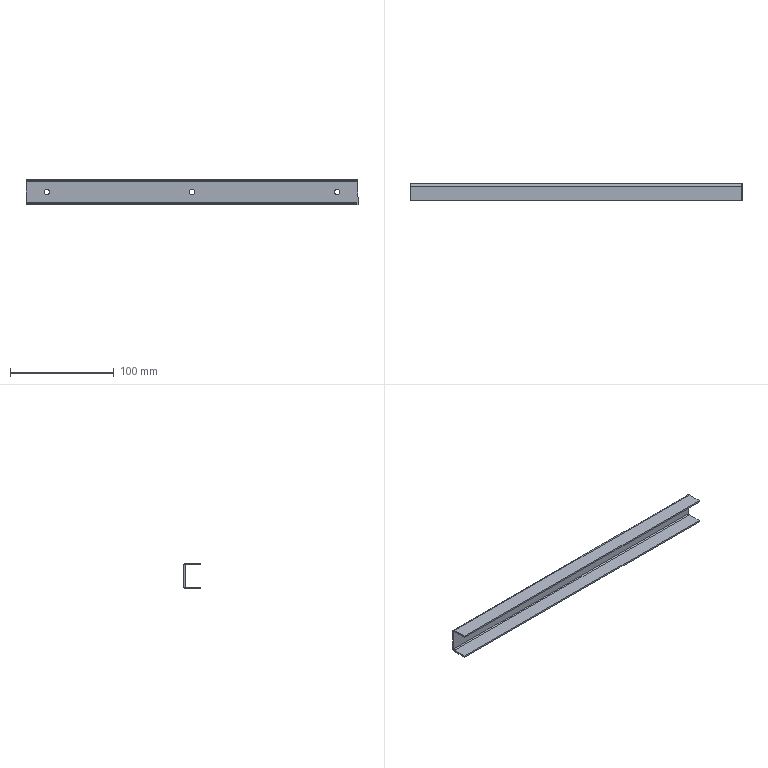Component | SolidWorks | GlassDoorAssembly-1_ShortBentPlate-5 | 1 solid | 28 faces | box 320 x 16 x 25 mm | volume 25103 mm3 | plane 18 | cylinder 10 | commonest cylinder face diameters 5.2 x6 5 x2 2 x2
STEP:
#1=CARTESIAN_POINT('',(-2.487,-19.472,-59.39));
#2=VERTEX_POINT('',#1);
#3=CARTESIAN_POINT('',(-2.283,-19.472,-59.39));
#4=VERTEX_POINT('',#3);
#5=CARTESIAN_POINT('',(-2.385,-19.472,-59.39));
#6=DIRECTION('',(0.,-1.,0.));
#7=DIRECTION('',(1.,0.,0.));
#8=AXIS2_PLACEMENT_3D('',#5,#6,#7);
#9=CIRCLE('',#8,0.1024);
#10=EDGE_CURVE('',#2,#4,#9,.T.);
#11=ORIENTED_EDGE('',*,*,#10,.T.);
#12=CARTESIAN_POINT('',(-2.283,-19.412,-59.39));
#13=VERTEX_POINT('',#12);
#14=CARTESIAN_POINT('',(-2.283,-19.491,-59.39));
#15=DIRECTION('',(-0.,1.,-0.));
#16=VECTOR('',#15,39.37);
#17=LINE('',#14,#16);
#18=EDGE_CURVE('',#4,#13,#17,.T.);
#19=ORIENTED_EDGE('',*,*,#18,.T.);
#20=CARTESIAN_POINT('',(-2.487,-19.412,-59.39));
#21=VERTEX_POINT('',#20);
#22=CARTESIAN_POINT('',(-2.385,-19.412,-59.39));
#23=DIRECTION('',(-0.,1.,-0.));
#24=DIRECTION('',(-1.,0.,0.));
#25=AXIS2_PLACEMENT_3D('',#22,#23,#24);
#26=CIRCLE('',#25,0.1024);
#27=EDGE_CURVE('',#13,#21,#26,.T.);
#28=ORIENTED_EDGE('',*,*,#27,.T.);
#29=CARTESIAN_POINT('',(-2.487,-19.491,-59.39));
#30=DIRECTION('',(-0.,1.,-0.));
#31=VECTOR('',#30,39.37);
#32=LINE('',#29,#31);
#33=EDGE_CURVE('',#2,#21,#32,.T.);
#34=ORIENTED_EDGE('',*,*,#33,.F.);
#35=EDGE_LOOP('',(#11,#19,#28,#34));
#36=FACE_OUTER_BOUND('',#35,.T.);
#37=CARTESIAN_POINT('',(-2.385,-19.491,-59.39));
#38=DIRECTION('',(-0.,1.,-0.));
#39=DIRECTION('',(-1.,0.,0.));
#40=AXIS2_PLACEMENT_3D('',#37,#38,#39);
#41=CYLINDRICAL_SURFACE('',#40,0.1024);
#42=ADVANCED_FACE('',(#36),#41,.F.);
#43=CARTESIAN_POINT('',(-13.511,-19.472,-59.39));
#44=VERTEX_POINT('',#43);
#45=CARTESIAN_POINT('',(-13.306,-19.472,-59.39));
#46=VERTEX_POINT('',#45);
#47=CARTESIAN_POINT('',(-13.409,-19.472,-59.39));
#48=DIRECTION('',(0.,-1.,0.));
#49=DIRECTION('',(1.,0.,0.));
#50=AXIS2_PLACEMENT_3D('',#47,#48,#49);
#51=CIRCLE('',#50,0.1024);
#52=EDGE_CURVE('',#44,#46,#51,.T.);
#53=ORIENTED_EDGE('',*,*,#52,.T.);
#54=CARTESIAN_POINT('',(-13.306,-19.412,-59.39));
#55=VERTEX_POINT('',#54);
#56=CARTESIAN_POINT('',(-13.306,-19.491,-59.39));
#57=DIRECTION('',(-0.,1.,-0.));
#58=VECTOR('',#57,39.37);
#59=LINE('',#56,#58);
#60=EDGE_CURVE('',#46,#55,#59,.T.);
#61=ORIENTED_EDGE('',*,*,#60,.T.);
#62=CARTESIAN_POINT('',(-13.511,-19.412,-59.39));
#63=VERTEX_POINT('',#62);
#64=CARTESIAN_POINT('',(-13.409,-19.412,-59.39));
#65=DIRECTION('',(-0.,1.,-0.));
#66=DIRECTION('',(-1.,0.,0.));
#67=AXIS2_PLACEMENT_3D('',#64,#65,#66);
#68=CIRCLE('',#67,0.1024);
#69=EDGE_CURVE('',#55,#63,#68,.T.);
#70=ORIENTED_EDGE('',*,*,#69,.T.);
#71=CARTESIAN_POINT('',(-13.511,-19.491,-59.39));
#72=DIRECTION('',(-0.,1.,-0.));
#73=VECTOR('',#72,39.37);
#74=LINE('',#71,#73);
#75=EDGE_CURVE('',#44,#63,#74,.T.);
#76=ORIENTED_EDGE('',*,*,#75,.F.);
#77=EDGE_LOOP('',(#53,#61,#70,#76));
#78=FACE_OUTER_BOUND('',#77,.T.);
#79=CARTESIAN_POINT('',(-13.409,-19.491,-59.39));
#80=DIRECTION('',(-0.,1.,-0.));
#81=DIRECTION('',(-1.,0.,0.));
#82=AXIS2_PLACEMENT_3D('',#79,#80,#81);
#83=CYLINDRICAL_SURFACE('',#82,0.1024);
#84=ADVANCED_FACE('',(#78),#83,.F.);
#85=CARTESIAN_POINT('',(-7.999,-19.472,-59.39));
#86=VERTEX_POINT('',#85);
#87=CARTESIAN_POINT('',(-7.794,-19.472,-59.39));
#88=VERTEX_POINT('',#87);
#89=CARTESIAN_POINT('',(-7.897,-19.472,-59.39));
#90=DIRECTION('',(0.,-1.,0.));
#91=DIRECTION('',(1.,0.,0.));
#92=AXIS2_PLACEMENT_3D('',#89,#90,#91);
#93=CIRCLE('',#92,0.1024);
#94=EDGE_CURVE('',#86,#88,#93,.T.);
#95=ORIENTED_EDGE('',*,*,#94,.T.);
#96=CARTESIAN_POINT('',(-7.794,-19.412,-59.39));
#97=VERTEX_POINT('',#96);
#98=CARTESIAN_POINT('',(-7.794,-19.491,-59.39));
#99=DIRECTION('',(-0.,1.,-0.));
#100=VECTOR('',#99,39.37);
#101=LINE('',#98,#100);
#102=EDGE_CURVE('',#88,#97,#101,.T.);
#103=ORIENTED_EDGE('',*,*,#102,.T.);
#104=CARTESIAN_POINT('',(-7.999,-19.412,-59.39));
#105=VERTEX_POINT('',#104);
#106=CARTESIAN_POINT('',(-7.897,-19.412,-59.39));
#107=DIRECTION('',(-0.,1.,-0.));
#108=DIRECTION('',(-1.,0.,0.));
#109=AXIS2_PLACEMENT_3D('',#106,#107,#108);
#110=CIRCLE('',#109,0.1024);
#111=EDGE_CURVE('',#97,#105,#110,.T.);
#112=ORIENTED_EDGE('',*,*,#111,.T.);
#113=CARTESIAN_POINT('',(-7.999,-19.491,-59.39));
#114=DIRECTION('',(-0.,1.,-0.));
#115=VECTOR('',#114,39.37);
#116=LINE('',#113,#115);
#117=EDGE_CURVE('',#86,#105,#116,.T.);
#118=ORIENTED_EDGE('',*,*,#117,.F.);
#119=EDGE_LOOP('',(#95,#103,#112,#118));
#120=FACE_OUTER_BOUND('',#119,.T.);
#121=CARTESIAN_POINT('',(-7.897,-19.491,-59.39));
#122=DIRECTION('',(-0.,1.,-0.));
#123=DIRECTION('',(-1.,0.,0.));
#124=AXIS2_PLACEMENT_3D('',#121,#122,#123);
#125=CYLINDRICAL_SURFACE('',#124,0.1024);
#126=ADVANCED_FACE('',(#120),#125,.F.);
#127=CARTESIAN_POINT('',(-2.385,-19.412,-59.39));
#128=DIRECTION('',(-0.,1.,-0.));
#129=DIRECTION('',(-1.,0.,0.));
#130=AXIS2_PLACEMENT_3D('',#127,#128,#129);
#131=CIRCLE('',#130,0.1024);
#132=EDGE_CURVE('',#21,#13,#131,.T.);
#133=ORIENTED_EDGE('',*,*,#132,.F.);
#134=ORIENTED_EDGE('',*,*,#27,.F.);
#135=EDGE_LOOP('',(#133,#134));
#136=FACE_BOUND('',#135,.T.);
#137=CARTESIAN_POINT('',(-13.409,-19.412,-59.39));
#138=DIRECTION('',(-0.,1.,-0.));
#139=DIRECTION('',(-1.,0.,0.));
#140=AXIS2_PLACEMENT_3D('',#137,#138,#139);
#141=CIRCLE('',#140,0.1024);
#142=EDGE_CURVE('',#63,#55,#141,.T.);
#143=ORIENTED_EDGE('',*,*,#142,.F.);
#144=ORIENTED_EDGE('',*,*,#69,.F.);
#145=EDGE_LOOP('',(#143,#144));
#146=FACE_BOUND('',#145,.T.);
#147=CARTESIAN_POINT('',(-7.897,-19.412,-59.39));
#148=DIRECTION('',(-0.,1.,-0.));
#149=DIRECTION('',(-1.,0.,0.));
#150=AXIS2_PLACEMENT_3D('',#147,#148,#149);
#151=CIRCLE('',#150,0.1024);
#152=EDGE_CURVE('',#105,#97,#151,.T.);
#153=ORIENTED_EDGE('',*,*,#152,.F.);
#154=ORIENTED_EDGE('',*,*,#111,.F.);
#155=EDGE_LOOP('',(#153,#154));
#156=FACE_BOUND('',#155,.T.);
#157=CARTESIAN_POINT('',(-14.196,-19.412,-58.996));
#158=VERTEX_POINT('',#157);
#159=CARTESIAN_POINT('',(-1.598,-19.412,-58.996));
#160=VERTEX_POINT('',#159);
#161=CARTESIAN_POINT('',(-14.196,-19.412,-58.996));
#162=DIRECTION('',(1.,0.,0.));
#163=VECTOR('',#162,39.37);
#164=LINE('',#161,#163);
#165=EDGE_CURVE('',#158,#160,#164,.T.);
#166=ORIENTED_EDGE('',*,*,#165,.T.);
#167=CARTESIAN_POINT('',(-1.598,-19.412,-59.783));
#168=VERTEX_POINT('',#167);
#169=CARTESIAN_POINT('',(-1.598,-19.412,-58.898));
#170=DIRECTION('',(-0.,0.,1.));
#171=VECTOR('',#170,39.37);
#172=LINE('',#169,#171);
#173=EDGE_CURVE('',#168,#160,#172,.T.);
#174=ORIENTED_EDGE('',*,*,#173,.F.);
#175=CARTESIAN_POINT('',(-14.196,-19.412,-59.783));
#176=VERTEX_POINT('',#175);
#177=CARTESIAN_POINT('',(-1.598,-19.412,-59.783));
#178=DIRECTION('',(-1.,-0.,-0.));
#179=VECTOR('',#178,39.37);
#180=LINE('',#177,#179);
#181=EDGE_CURVE('',#168,#176,#180,.T.);
#182=ORIENTED_EDGE('',*,*,#181,.T.);
#183=CARTESIAN_POINT('',(-14.196,-19.412,-58.898));
#184=DIRECTION('',(0.,-0.,-1.));
#185=VECTOR('',#184,39.37);
#186=LINE('',#183,#185);
#187=EDGE_CURVE('',#158,#176,#186,.T.);
#188=ORIENTED_EDGE('',*,*,#187,.F.);
#189=EDGE_LOOP('',(#166,#174,#182,#188));
#190=FACE_OUTER_BOUND('',#189,.T.);
#191=CARTESIAN_POINT('',(-1.598,-19.412,-59.882));
#192=DIRECTION('',(0.,-1.,0.));
#193=DIRECTION('',(1.,0.,0.));
#194=AXIS2_PLACEMENT_3D('',#191,#192,#193);
#195=PLANE('',#194);
#196=ADVANCED_FACE('',(#136,#146,#156,#190),#195,.F.);
#197=ORIENTED_EDGE('',*,*,#10,.F.);
#198=CARTESIAN_POINT('',(-2.385,-19.472,-59.39));
#199=DIRECTION('',(0.,-1.,0.));
#200=DIRECTION('',(1.,0.,0.));
#201=AXIS2_PLACEMENT_3D('',#198,#199,#200);
#202=CIRCLE('',#201,0.1024);
#203=EDGE_CURVE('',#4,#2,#202,.T.);
#204=ORIENTED_EDGE('',*,*,#203,.F.);
#205=EDGE_LOOP('',(#197,#204));
#206=FACE_BOUND('',#205,.T.);
#207=ORIENTED_EDGE('',*,*,#52,.F.);
#208=CARTESIAN_POINT('',(-13.409,-19.472,-59.39));
#209=DIRECTION('',(0.,-1.,0.));
#210=DIRECTION('',(1.,0.,0.));
#211=AXIS2_PLACEMENT_3D('',#208,#209,#210);
#212=CIRCLE('',#211,0.1024);
#213=EDGE_CURVE('',#46,#44,#212,.T.);
#214=ORIENTED_EDGE('',*,*,#213,.F.);
#215=EDGE_LOOP('',(#207,#214));
#216=FACE_BOUND('',#215,.T.);
#217=ORIENTED_EDGE('',*,*,#94,.F.);
#218=CARTESIAN_POINT('',(-7.897,-19.472,-59.39));
#219=DIRECTION('',(0.,-1.,0.));
#220=DIRECTION('',(1.,0.,0.));
#221=AXIS2_PLACEMENT_3D('',#218,#219,#220);
#222=CIRCLE('',#221,0.1024);
#223=EDGE_CURVE('',#88,#86,#222,.T.);
#224=ORIENTED_EDGE('',*,*,#223,.F.);
#225=EDGE_LOOP('',(#217,#224));
#226=FACE_BOUND('',#225,.T.);
#227=CARTESIAN_POINT('',(-1.598,-19.472,-59.783));
#228=VERTEX_POINT('',#227);
#229=CARTESIAN_POINT('',(-1.598,-19.472,-58.996));
#230=VERTEX_POINT('',#229);
#231=CARTESIAN_POINT('',(-1.598,-19.472,-58.898));
#232=DIRECTION('',(-0.,0.,1.));
#233=VECTOR('',#232,39.37);
#234=LINE('',#231,#233);
#235=EDGE_CURVE('',#228,#230,#234,.T.);
#236=ORIENTED_EDGE('',*,*,#235,.T.);
#237=CARTESIAN_POINT('',(-14.196,-19.472,-58.996));
#238=VERTEX_POINT('',#237);
#239=CARTESIAN_POINT('',(-14.196,-19.472,-58.996));
#240=DIRECTION('',(1.,0.,0.));
#241=VECTOR('',#240,39.37);
#242=LINE('',#239,#241);
#243=EDGE_CURVE('',#238,#230,#242,.T.);
#244=ORIENTED_EDGE('',*,*,#243,.F.);
#245=CARTESIAN_POINT('',(-14.196,-19.472,-59.783));
#246=VERTEX_POINT('',#245);
#247=CARTESIAN_POINT('',(-14.196,-19.472,-58.898));
#248=DIRECTION('',(0.,-0.,-1.));
#249=VECTOR('',#248,39.37);
#250=LINE('',#247,#249);
#251=EDGE_CURVE('',#238,#246,#250,.T.);
#252=ORIENTED_EDGE('',*,*,#251,.T.);
#253=CARTESIAN_POINT('',(-1.598,-19.472,-59.783));
#254=DIRECTION('',(-1.,-0.,-0.));
#255=VECTOR('',#254,39.37);
#256=LINE('',#253,#255);
#257=EDGE_CURVE('',#228,#246,#256,.T.);
#258=ORIENTED_EDGE('',*,*,#257,.F.);
#259=EDGE_LOOP('',(#236,#244,#252,#258));
#260=FACE_OUTER_BOUND('',#259,.T.);
#261=CARTESIAN_POINT('',(-1.598,-19.472,-59.882));
#262=DIRECTION('',(0.,-1.,0.));
#263=DIRECTION('',(1.,0.,0.));
#264=AXIS2_PLACEMENT_3D('',#261,#262,#263);
#265=PLANE('',#264);
#266=ADVANCED_FACE('',(#206,#216,#226,#260),#265,.T.);
#267=ORIENTED_EDGE('',*,*,#251,.F.);
#268=CARTESIAN_POINT('',(-14.196,-19.472,-58.996));
#269=DIRECTION('',(-0.,1.,-0.));
#270=VECTOR('',#269,39.37);
#271=LINE('',#268,#270);
#272=EDGE_CURVE('',#238,#158,#271,.T.);
#273=ORIENTED_EDGE('',*,*,#272,.T.);
#274=ORIENTED_EDGE('',*,*,#187,.T.);
#275=CARTESIAN_POINT('',(-14.196,-19.472,-59.783));
#276=DIRECTION('',(-0.,1.,-0.));
#277=VECTOR('',#276,39.37);
#278=LINE('',#275,#277);
#279=EDGE_CURVE('',#246,#176,#278,.T.);
#280=ORIENTED_EDGE('',*,*,#279,.F.);
#281=EDGE_LOOP('',(#267,#273,#274,#280));
#282=FACE_OUTER_BOUND('',#281,.T.);
#283=CARTESIAN_POINT('',(-14.196,-19.412,-58.898));
#284=DIRECTION('',(-1.,-0.,-0.));
#285=DIRECTION('',(0.,-1.,0.));
#286=AXIS2_PLACEMENT_3D('',#283,#284,#285);
#287=PLANE('',#286);
#288=ADVANCED_FACE('',(#282),#287,.T.);
#289=CARTESIAN_POINT('',(-1.598,-19.472,-58.996));
#290=DIRECTION('',(-0.,1.,-0.));
#291=VECTOR('',#290,39.37);
#292=LINE('',#289,#291);
#293=EDGE_CURVE('',#230,#160,#292,.T.);
#294=ORIENTED_EDGE('',*,*,#293,.F.);
#295=ORIENTED_EDGE('',*,*,#235,.F.);
#296=CARTESIAN_POINT('',(-1.598,-19.472,-59.783));
#297=DIRECTION('',(-0.,1.,-0.));
#298=VECTOR('',#297,39.37);
#299=LINE('',#296,#298);
#300=EDGE_CURVE('',#228,#168,#299,.T.);
#301=ORIENTED_EDGE('',*,*,#300,.T.);
#302=ORIENTED_EDGE('',*,*,#173,.T.);
#303=EDGE_LOOP('',(#294,#295,#301,#302));
#304=FACE_OUTER_BOUND('',#303,.T.);
#305=CARTESIAN_POINT('',(-1.598,-19.412,-58.898));
#306=DIRECTION('',(1.,0.,0.));
#307=DIRECTION('',(-0.,1.,-0.));
#308=AXIS2_PLACEMENT_3D('',#305,#306,#307);
#309=PLANE('',#308);
#310=ADVANCED_FACE('',(#304),#309,.T.);
#311=CARTESIAN_POINT('',(-14.196,-19.511,-59.823));
#312=VERTEX_POINT('',#311);
#313=CARTESIAN_POINT('',(-14.196,-19.511,-59.882));
#314=VERTEX_POINT('',#313);
#315=CARTESIAN_POINT('',(-14.196,-19.511,-59.882));
#316=DIRECTION('',(0.,0.,-1.));
#317=VECTOR('',#316,39.37);
#318=LINE('',#315,#317);
#319=EDGE_CURVE('',#312,#314,#318,.T.);
#320=ORIENTED_EDGE('',*,*,#319,.F.);
#321=CARTESIAN_POINT('',(-14.196,-19.511,-59.783));
#322=DIRECTION('',(-1.,-0.,-0.));
#323=DIRECTION('',(0.,1.,0.));
#324=AXIS2_PLACEMENT_3D('',#321,#322,#323);
#325=CIRCLE('',#324,0.03937);
#326=EDGE_CURVE('',#246,#312,#325,.T.);
#327=ORIENTED_EDGE('',*,*,#326,.F.);
#328=ORIENTED_EDGE('',*,*,#279,.T.);
#329=CARTESIAN_POINT('',(-14.196,-19.511,-59.783));
#330=DIRECTION('',(-1.,-0.,-0.));
#331=DIRECTION('',(0.,1.,0.));
#332=AXIS2_PLACEMENT_3D('',#329,#330,#331);
#333=CIRCLE('',#332,0.09843);
#334=EDGE_CURVE('',#176,#314,#333,.T.);
#335=ORIENTED_EDGE('',*,*,#334,.T.);
#336=EDGE_LOOP('',(#320,#327,#328,#335));
#337=FACE_OUTER_BOUND('',#336,.T.);
#338=CARTESIAN_POINT('',(-14.196,-19.511,-59.783));
#339=DIRECTION('',(-1.,-0.,-0.));
#340=DIRECTION('',(0.,-1.,0.));
#341=AXIS2_PLACEMENT_3D('',#338,#339,#340);
#342=PLANE('',#341);
#343=ADVANCED_FACE('',(#337),#342,.T.);
#344=CARTESIAN_POINT('',(-1.598,-19.511,-59.823));
#345=VERTEX_POINT('',#344);
#346=CARTESIAN_POINT('',(-1.598,-19.511,-59.783));
#347=DIRECTION('',(1.,0.,0.));
#348=DIRECTION('',(0.,1.,0.));
#349=AXIS2_PLACEMENT_3D('',#346,#347,#348);
#350=CIRCLE('',#349,0.03937);
#351=EDGE_CURVE('',#345,#228,#350,.T.);
#352=ORIENTED_EDGE('',*,*,#351,.F.);
#353=CARTESIAN_POINT('',(-1.598,-19.511,-59.882));
#354=VERTEX_POINT('',#353);
#355=CARTESIAN_POINT('',(-1.598,-19.511,-59.823));
#356=DIRECTION('',(0.,0.,-1.));
#357=VECTOR('',#356,39.37);
#358=LINE('',#355,#357);
#359=EDGE_CURVE('',#345,#354,#358,.T.);
#360=ORIENTED_EDGE('',*,*,#359,.T.);
#361=CARTESIAN_POINT('',(-1.598,-19.511,-59.783));
#362=DIRECTION('',(1.,0.,0.));
#363=DIRECTION('',(0.,1.,0.));
#364=AXIS2_PLACEMENT_3D('',#361,#362,#363);
#365=CIRCLE('',#364,0.09843);
#366=EDGE_CURVE('',#354,#168,#365,.T.);
#367=ORIENTED_EDGE('',*,*,#366,.T.);
#368=ORIENTED_EDGE('',*,*,#300,.F.);
#369=EDGE_LOOP('',(#352,#360,#367,#368));
#370=FACE_OUTER_BOUND('',#369,.T.);
#371=CARTESIAN_POINT('',(-1.598,-19.511,-59.783));
#372=DIRECTION('',(-1.,-0.,-0.));
#373=DIRECTION('',(0.,-1.,0.));
#374=AXIS2_PLACEMENT_3D('',#371,#372,#373);
#375=PLANE('',#374);
#376=ADVANCED_FACE('',(#370),#375,.F.);
#377=ORIENTED_EDGE('',*,*,#181,.F.);
#378=ORIENTED_EDGE('',*,*,#366,.F.);
#379=CARTESIAN_POINT('',(-14.196,-19.511,-59.882));
#380=DIRECTION('',(-1.,-0.,-0.));
#381=VECTOR('',#380,39.37);
#382=LINE('',#379,#381);
#383=EDGE_CURVE('',#354,#314,#382,.T.);
#384=ORIENTED_EDGE('',*,*,#383,.T.);
#385=ORIENTED_EDGE('',*,*,#334,.F.);
#386=EDGE_LOOP('',(#377,#378,#384,#385));
#387=FACE_OUTER_BOUND('',#386,.T.);
#388=CARTESIAN_POINT('',(-1.598,-19.511,-59.783));
#389=DIRECTION('',(1.,0.,0.));
#390=DIRECTION('',(0.,0.,-1.));
#391=AXIS2_PLACEMENT_3D('',#388,#389,#390);
#392=CYLINDRICAL_SURFACE('',#391,0.09843);
#393=ADVANCED_FACE('',(#387),#392,.T.);
#394=ORIENTED_EDGE('',*,*,#257,.T.);
#395=ORIENTED_EDGE('',*,*,#326,.T.);
#396=CARTESIAN_POINT('',(-14.196,-19.511,-59.823));
#397=DIRECTION('',(1.,0.,0.));
#398=VECTOR('',#397,39.37);
#399=LINE('',#396,#398);
#400=EDGE_CURVE('',#312,#345,#399,.T.);
#401=ORIENTED_EDGE('',*,*,#400,.T.);
#402=ORIENTED_EDGE('',*,*,#351,.T.);
#403=EDGE_LOOP('',(#394,#395,#401,#402));
#404=FACE_OUTER_BOUND('',#403,.T.);
#405=CARTESIAN_POINT('',(-1.598,-19.511,-59.783));
#406=DIRECTION('',(1.,0.,0.));
#407=DIRECTION('',(0.,0.,-1.));
#408=AXIS2_PLACEMENT_3D('',#405,#406,#407);
#409=CYLINDRICAL_SURFACE('',#408,0.03937);
#410=ADVANCED_FACE('',(#404),#409,.F.);
#411=ORIENTED_EDGE('',*,*,#319,.T.);
#412=CARTESIAN_POINT('',(-14.196,-20.042,-59.882));
#413=VERTEX_POINT('',#412);
#414=CARTESIAN_POINT('',(-14.196,-20.042,-59.882));
#415=DIRECTION('',(-0.,1.,0.));
#416=VECTOR('',#415,39.37);
#417=LINE('',#414,#416);
#418=EDGE_CURVE('',#413,#314,#417,.T.);
#419=ORIENTED_EDGE('',*,*,#418,.F.);
#420=CARTESIAN_POINT('',(-14.196,-20.042,-59.823));
#421=VERTEX_POINT('',#420);
#422=CARTESIAN_POINT('',(-14.196,-20.042,-59.882));
#423=DIRECTION('',(-0.,-0.,1.));
#424=VECTOR('',#423,39.37);
#425=LINE('',#422,#424);
#426=EDGE_CURVE('',#413,#421,#425,.T.);
#427=ORIENTED_EDGE('',*,*,#426,.T.);
#428=CARTESIAN_POINT('',(-14.196,-19.472,-59.823));
#429=DIRECTION('',(-0.,1.,0.));
#430=VECTOR('',#429,39.37);
#431=LINE('',#428,#430);
#432=EDGE_CURVE('',#421,#312,#431,.T.);
#433=ORIENTED_EDGE('',*,*,#432,.T.);
#434=EDGE_LOOP('',(#411,#419,#427,#433));
#435=FACE_OUTER_BOUND('',#434,.T.);
#436=CARTESIAN_POINT('',(-14.196,-19.472,-59.882));
#437=DIRECTION('',(1.,0.,0.));
#438=DIRECTION('',(-0.,1.,-0.));
#439=AXIS2_PLACEMENT_3D('',#436,#437,#438);
#440=PLANE('',#439);
#441=ADVANCED_FACE('',(#435),#440,.F.);
#442=ORIENTED_EDGE('',*,*,#359,.F.);
#443=CARTESIAN_POINT('',(-1.598,-20.042,-59.823));
#444=VERTEX_POINT('',#443);
#445=CARTESIAN_POINT('',(-1.598,-20.042,-59.823));
#446=DIRECTION('',(0.,-1.,-0.));
#447=VECTOR('',#446,39.37);
#448=LINE('',#445,#447);
#449=EDGE_CURVE('',#345,#444,#448,.T.);
#450=ORIENTED_EDGE('',*,*,#449,.T.);
#451=CARTESIAN_POINT('',(-1.598,-20.042,-59.882));
#452=VERTEX_POINT('',#451);
#453=CARTESIAN_POINT('',(-1.598,-20.042,-59.882));
#454=DIRECTION('',(-0.,-0.,1.));
#455=VECTOR('',#454,39.37);
#456=LINE('',#453,#455);
#457=EDGE_CURVE('',#452,#444,#456,.T.);
#458=ORIENTED_EDGE('',*,*,#457,.F.);
#459=CARTESIAN_POINT('',(-1.598,-20.042,-59.882));
#460=DIRECTION('',(0.,-1.,-0.));
#461=VECTOR('',#460,39.37);
#462=LINE('',#459,#461);
#463=EDGE_CURVE('',#354,#452,#462,.T.);
#464=ORIENTED_EDGE('',*,*,#463,.F.);
#465=EDGE_LOOP('',(#442,#450,#458,#464));
#466=FACE_OUTER_BOUND('',#465,.T.);
#467=CARTESIAN_POINT('',(-1.598,-20.042,-59.882));
#468=DIRECTION('',(-1.,-0.,-0.));
#469=DIRECTION('',(0.,-1.,0.));
#470=AXIS2_PLACEMENT_3D('',#467,#468,#469);
#471=PLANE('',#470);
#472=ADVANCED_FACE('',(#466),#471,.F.);
#473=ORIENTED_EDGE('',*,*,#383,.F.);
#474=ORIENTED_EDGE('',*,*,#463,.T.);
#475=CARTESIAN_POINT('',(-14.196,-20.042,-59.882));
#476=DIRECTION('',(-1.,-0.,-0.));
#477=VECTOR('',#476,39.37);
#478=LINE('',#475,#477);
#479=EDGE_CURVE('',#452,#413,#478,.T.);
#480=ORIENTED_EDGE('',*,*,#479,.T.);
#481=ORIENTED_EDGE('',*,*,#418,.T.);
#482=EDGE_LOOP('',(#473,#474,#480,#481));
#483=FACE_OUTER_BOUND('',#482,.T.);
#484=CARTESIAN_POINT('',(-14.196,-20.042,-59.882));
#485=DIRECTION('',(-0.,-0.,1.));
#486=DIRECTION('',(0.,-1.,-0.));
#487=AXIS2_PLACEMENT_3D('',#484,#485,#486);
#488=PLANE('',#487);
#489=ADVANCED_FACE('',(#483),#488,.F.);
#490=ORIENTED_EDGE('',*,*,#449,.F.);
#491=ORIENTED_EDGE('',*,*,#400,.F.);
#492=ORIENTED_EDGE('',*,*,#432,.F.);
#493=CARTESIAN_POINT('',(-14.196,-20.042,-59.823));
#494=DIRECTION('',(-1.,-0.,-0.));
#495=VECTOR('',#494,39.37);
#496=LINE('',#493,#495);
#497=EDGE_CURVE('',#444,#421,#496,.T.);
#498=ORIENTED_EDGE('',*,*,#497,.F.);
#499=EDGE_LOOP('',(#490,#491,#492,#498));
#500=FACE_OUTER_BOUND('',#499,.T.);
#501=CARTESIAN_POINT('',(-14.196,-20.042,-59.823));
#502=DIRECTION('',(-0.,-0.,1.));
#503=DIRECTION('',(0.,-1.,-0.));
#504=AXIS2_PLACEMENT_3D('',#501,#502,#503);
#505=PLANE('',#504);
#506=ADVANCED_FACE('',(#500),#505,.T.);
#507=ORIENTED_EDGE('',*,*,#497,.T.);
#508=ORIENTED_EDGE('',*,*,#426,.F.);
#509=ORIENTED_EDGE('',*,*,#479,.F.);
#510=ORIENTED_EDGE('',*,*,#457,.T.);
#511=EDGE_LOOP('',(#507,#508,#509,#510));
#512=FACE_OUTER_BOUND('',#511,.T.);
#513=CARTESIAN_POINT('',(-14.196,-20.042,-59.882));
#514=DIRECTION('',(-0.,1.,0.));
#515=DIRECTION('',(-0.,-0.,1.));
#516=AXIS2_PLACEMENT_3D('',#513,#514,#515);
#517=PLANE('',#516);
#518=ADVANCED_FACE('',(#512),#517,.F.);
#519=CARTESIAN_POINT('',(-1.598,-19.511,-58.957));
#520=VERTEX_POINT('',#519);
#521=CARTESIAN_POINT('',(-1.598,-19.511,-58.898));
#522=VERTEX_POINT('',#521);
#523=CARTESIAN_POINT('',(-1.598,-19.511,-58.898));
#524=DIRECTION('',(-0.,0.,1.));
#525=VECTOR('',#524,39.37);
#526=LINE('',#523,#525);
#527=EDGE_CURVE('',#520,#522,#526,.T.);
#528=ORIENTED_EDGE('',*,*,#527,.F.);
#529=CARTESIAN_POINT('',(-1.598,-19.511,-58.996));
#530=DIRECTION('',(1.,0.,0.));
#531=DIRECTION('',(0.,-1.,0.));
#532=AXIS2_PLACEMENT_3D('',#529,#530,#531);
#533=CIRCLE('',#532,0.03937);
#534=EDGE_CURVE('',#230,#520,#533,.T.);
#535=ORIENTED_EDGE('',*,*,#534,.F.);
#536=ORIENTED_EDGE('',*,*,#293,.T.);
#537=CARTESIAN_POINT('',(-1.598,-19.511,-58.996));
#538=DIRECTION('',(1.,0.,0.));
#539=DIRECTION('',(0.,-1.,0.));
#540=AXIS2_PLACEMENT_3D('',#537,#538,#539);
#541=CIRCLE('',#540,0.09843);
#542=EDGE_CURVE('',#160,#522,#541,.T.);
#543=ORIENTED_EDGE('',*,*,#542,.T.);
#544=EDGE_LOOP('',(#528,#535,#536,#543));
#545=FACE_OUTER_BOUND('',#544,.T.);
#546=CARTESIAN_POINT('',(-1.598,-19.511,-58.996));
#547=DIRECTION('',(1.,0.,0.));
#548=DIRECTION('',(-0.,1.,-0.));
#549=AXIS2_PLACEMENT_3D('',#546,#547,#548);
#550=PLANE('',#549);
#551=ADVANCED_FACE('',(#545),#550,.T.);
#552=CARTESIAN_POINT('',(-14.196,-19.511,-58.957));
#553=VERTEX_POINT('',#552);
#554=CARTESIAN_POINT('',(-14.196,-19.511,-58.996));
#555=DIRECTION('',(-1.,-0.,-0.));
#556=DIRECTION('',(0.,-1.,0.));
#557=AXIS2_PLACEMENT_3D('',#554,#555,#556);
#558=CIRCLE('',#557,0.03937);
#559=EDGE_CURVE('',#553,#238,#558,.T.);
#560=ORIENTED_EDGE('',*,*,#559,.F.);
#561=CARTESIAN_POINT('',(-14.196,-19.511,-58.898));
#562=VERTEX_POINT('',#561);
#563=CARTESIAN_POINT('',(-14.196,-19.511,-58.957));
#564=DIRECTION('',(-0.,0.,1.));
#565=VECTOR('',#564,39.37);
#566=LINE('',#563,#565);
#567=EDGE_CURVE('',#553,#562,#566,.T.);
#568=ORIENTED_EDGE('',*,*,#567,.T.);
#569=CARTESIAN_POINT('',(-14.196,-19.511,-58.996));
#570=DIRECTION('',(-1.,-0.,-0.));
#571=DIRECTION('',(0.,-1.,0.));
#572=AXIS2_PLACEMENT_3D('',#569,#570,#571);
#573=CIRCLE('',#572,0.09843);
#574=EDGE_CURVE('',#562,#158,#573,.T.);
#575=ORIENTED_EDGE('',*,*,#574,.T.);
#576=ORIENTED_EDGE('',*,*,#272,.F.);
#577=EDGE_LOOP('',(#560,#568,#575,#576));
#578=FACE_OUTER_BOUND('',#577,.T.);
#579=CARTESIAN_POINT('',(-14.196,-19.511,-58.996));
#580=DIRECTION('',(1.,0.,0.));
#581=DIRECTION('',(-0.,1.,-0.));
#582=AXIS2_PLACEMENT_3D('',#579,#580,#581);
#583=PLANE('',#582);
#584=ADVANCED_FACE('',(#578),#583,.F.);
#585=ORIENTED_EDGE('',*,*,#165,.F.);
#586=ORIENTED_EDGE('',*,*,#574,.F.);
#587=CARTESIAN_POINT('',(-1.598,-19.511,-58.898));
#588=DIRECTION('',(1.,0.,0.));
#589=VECTOR('',#588,39.37);
#590=LINE('',#587,#589);
#591=EDGE_CURVE('',#562,#522,#590,.T.);
#592=ORIENTED_EDGE('',*,*,#591,.T.);
#593=ORIENTED_EDGE('',*,*,#542,.F.);
#594=EDGE_LOOP('',(#585,#586,#592,#593));
#595=FACE_OUTER_BOUND('',#594,.T.);
#596=CARTESIAN_POINT('',(-14.196,-19.511,-58.996));
#597=DIRECTION('',(-1.,-0.,-0.));
#598=DIRECTION('',(0.,0.,1.));
#599=AXIS2_PLACEMENT_3D('',#596,#597,#598);
#600=CYLINDRICAL_SURFACE('',#599,0.09843);
#601=ADVANCED_FACE('',(#595),#600,.T.);
#602=ORIENTED_EDGE('',*,*,#243,.T.);
#603=ORIENTED_EDGE('',*,*,#534,.T.);
#604=CARTESIAN_POINT('',(-1.598,-19.511,-58.957));
#605=DIRECTION('',(-1.,-0.,-0.));
#606=VECTOR('',#605,39.37);
#607=LINE('',#604,#606);
#608=EDGE_CURVE('',#520,#553,#607,.T.);
#609=ORIENTED_EDGE('',*,*,#608,.T.);
#610=ORIENTED_EDGE('',*,*,#559,.T.);
#611=EDGE_LOOP('',(#602,#603,#609,#610));
#612=FACE_OUTER_BOUND('',#611,.T.);
#613=CARTESIAN_POINT('',(-14.196,-19.511,-58.996));
#614=DIRECTION('',(-1.,-0.,-0.));
#615=DIRECTION('',(0.,0.,1.));
#616=AXIS2_PLACEMENT_3D('',#613,#614,#615);
#617=CYLINDRICAL_SURFACE('',#616,0.03937);
#618=ADVANCED_FACE('',(#612),#617,.F.);
#619=ORIENTED_EDGE('',*,*,#527,.T.);
#620=CARTESIAN_POINT('',(-1.598,-20.042,-58.898));
#621=VERTEX_POINT('',#620);
#622=CARTESIAN_POINT('',(-1.598,-20.042,-58.898));
#623=DIRECTION('',(-0.,1.,-0.));
#624=VECTOR('',#623,39.37);
#625=LINE('',#622,#624);
#626=EDGE_CURVE('',#621,#522,#625,.T.);
#627=ORIENTED_EDGE('',*,*,#626,.F.);
#628=CARTESIAN_POINT('',(-1.598,-20.042,-58.957));
#629=VERTEX_POINT('',#628);
#630=CARTESIAN_POINT('',(-1.598,-20.042,-58.898));
#631=DIRECTION('',(0.,-0.,-1.));
#632=VECTOR('',#631,39.37);
#633=LINE('',#630,#632);
#634=EDGE_CURVE('',#621,#629,#633,.T.);
#635=ORIENTED_EDGE('',*,*,#634,.T.);
#636=CARTESIAN_POINT('',(-1.598,-19.472,-58.957));
#637=DIRECTION('',(-0.,1.,-0.));
#638=VECTOR('',#637,39.37);
#639=LINE('',#636,#638);
#640=EDGE_CURVE('',#629,#520,#639,.T.);
#641=ORIENTED_EDGE('',*,*,#640,.T.);
#642=EDGE_LOOP('',(#619,#627,#635,#641));
#643=FACE_OUTER_BOUND('',#642,.T.);
#644=CARTESIAN_POINT('',(-1.598,-19.472,-58.898));
#645=DIRECTION('',(-1.,-0.,-0.));
#646=DIRECTION('',(0.,-1.,0.));
#647=AXIS2_PLACEMENT_3D('',#644,#645,#646);
#648=PLANE('',#647);
#649=ADVANCED_FACE('',(#643),#648,.F.);
#650=ORIENTED_EDGE('',*,*,#567,.F.);
#651=CARTESIAN_POINT('',(-14.196,-20.042,-58.957));
#652=VERTEX_POINT('',#651);
#653=CARTESIAN_POINT('',(-14.196,-20.042,-58.957));
#654=DIRECTION('',(0.,-1.,0.));
#655=VECTOR('',#654,39.37);
#656=LINE('',#653,#655);
#657=EDGE_CURVE('',#553,#652,#656,.T.);
#658=ORIENTED_EDGE('',*,*,#657,.T.);
#659=CARTESIAN_POINT('',(-14.196,-20.042,-58.898));
#660=VERTEX_POINT('',#659);
#661=CARTESIAN_POINT('',(-14.196,-20.042,-58.898));
#662=DIRECTION('',(0.,-0.,-1.));
#663=VECTOR('',#662,39.37);
#664=LINE('',#661,#663);
#665=EDGE_CURVE('',#660,#652,#664,.T.);
#666=ORIENTED_EDGE('',*,*,#665,.F.);
#667=CARTESIAN_POINT('',(-14.196,-20.042,-58.898));
#668=DIRECTION('',(0.,-1.,0.));
#669=VECTOR('',#668,39.37);
#670=LINE('',#667,#669);
#671=EDGE_CURVE('',#562,#660,#670,.T.);
#672=ORIENTED_EDGE('',*,*,#671,.F.);
#673=EDGE_LOOP('',(#650,#658,#666,#672));
#674=FACE_OUTER_BOUND('',#673,.T.);
#675=CARTESIAN_POINT('',(-14.196,-20.042,-58.898));
#676=DIRECTION('',(1.,0.,0.));
#677=DIRECTION('',(-0.,1.,-0.));
#678=AXIS2_PLACEMENT_3D('',#675,#676,#677);
#679=PLANE('',#678);
#680=ADVANCED_FACE('',(#674),#679,.F.);
#681=ORIENTED_EDGE('',*,*,#591,.F.);
#682=ORIENTED_EDGE('',*,*,#671,.T.);
#683=CARTESIAN_POINT('',(-1.598,-20.042,-58.898));
#684=DIRECTION('',(1.,0.,0.));
#685=VECTOR('',#684,39.37);
#686=LINE('',#683,#685);
#687=EDGE_CURVE('',#660,#621,#686,.T.);
#688=ORIENTED_EDGE('',*,*,#687,.T.);
#689=ORIENTED_EDGE('',*,*,#626,.T.);
#690=EDGE_LOOP('',(#681,#682,#688,#689));
#691=FACE_OUTER_BOUND('',#690,.T.);
#692=CARTESIAN_POINT('',(-1.598,-20.042,-58.898));
#693=DIRECTION('',(0.,-0.,-1.));
#694=DIRECTION('',(-0.,1.,-0.));
#695=AXIS2_PLACEMENT_3D('',#692,#693,#694);
#696=PLANE('',#695);
#697=ADVANCED_FACE('',(#691),#696,.F.);
#698=ORIENTED_EDGE('',*,*,#657,.F.);
#699=ORIENTED_EDGE('',*,*,#608,.F.);
#700=ORIENTED_EDGE('',*,*,#640,.F.);
#701=CARTESIAN_POINT('',(-1.598,-20.042,-58.957));
#702=DIRECTION('',(1.,0.,0.));
#703=VECTOR('',#702,39.37);
#704=LINE('',#701,#703);
#705=EDGE_CURVE('',#652,#629,#704,.T.);
#706=ORIENTED_EDGE('',*,*,#705,.F.);
#707=EDGE_LOOP('',(#698,#699,#700,#706));
#708=FACE_OUTER_BOUND('',#707,.T.);
#709=CARTESIAN_POINT('',(-1.598,-20.042,-58.957));
#710=DIRECTION('',(0.,-0.,-1.));
#711=DIRECTION('',(-0.,1.,-0.));
#712=AXIS2_PLACEMENT_3D('',#709,#710,#711);
#713=PLANE('',#712);
#714=ADVANCED_FACE('',(#708),#713,.T.);
#715=ORIENTED_EDGE('',*,*,#705,.T.);
#716=ORIENTED_EDGE('',*,*,#634,.F.);
#717=ORIENTED_EDGE('',*,*,#687,.F.);
#718=ORIENTED_EDGE('',*,*,#665,.T.);
#719=EDGE_LOOP('',(#715,#716,#717,#718));
#720=FACE_OUTER_BOUND('',#719,.T.);
#721=CARTESIAN_POINT('',(-1.598,-20.042,-58.898));
#722=DIRECTION('',(-0.,1.,-0.));
#723=DIRECTION('',(-0.,0.,1.));
#724=AXIS2_PLACEMENT_3D('',#721,#722,#723);
#725=PLANE('',#724);
#726=ADVANCED_FACE('',(#720),#725,.F.);
#727=ORIENTED_EDGE('',*,*,#102,.F.);
#728=ORIENTED_EDGE('',*,*,#223,.T.);
#729=ORIENTED_EDGE('',*,*,#117,.T.);
#730=ORIENTED_EDGE('',*,*,#152,.T.);
#731=EDGE_LOOP('',(#727,#728,#729,#730));
#732=FACE_OUTER_BOUND('',#731,.T.);
#733=CARTESIAN_POINT('',(-7.897,-19.491,-59.39));
#734=DIRECTION('',(-0.,1.,-0.));
#735=DIRECTION('',(-1.,0.,0.));
#736=AXIS2_PLACEMENT_3D('',#733,#734,#735);
#737=CYLINDRICAL_SURFACE('',#736,0.1024);
#738=ADVANCED_FACE('',(#732),#737,.F.);
#739=ORIENTED_EDGE('',*,*,#60,.F.);
#740=ORIENTED_EDGE('',*,*,#213,.T.);
#741=ORIENTED_EDGE('',*,*,#75,.T.);
#742=ORIENTED_EDGE('',*,*,#142,.T.);
#743=EDGE_LOOP('',(#739,#740,#741,#742));
#744=FACE_OUTER_BOUND('',#743,.T.);
#745=CARTESIAN_POINT('',(-13.409,-19.491,-59.39));
#746=DIRECTION('',(-0.,1.,-0.));
#747=DIRECTION('',(-1.,0.,0.));
#748=AXIS2_PLACEMENT_3D('',#745,#746,#747);
#749=CYLINDRICAL_SURFACE('',#748,0.1024);
#750=ADVANCED_FACE('',(#744),#749,.F.);
#751=ORIENTED_EDGE('',*,*,#18,.F.);
#752=ORIENTED_EDGE('',*,*,#203,.T.);
#753=ORIENTED_EDGE('',*,*,#33,.T.);
#754=ORIENTED_EDGE('',*,*,#132,.T.);
#755=EDGE_LOOP('',(#751,#752,#753,#754));
#756=FACE_OUTER_BOUND('',#755,.T.);
#757=CARTESIAN_POINT('',(-2.385,-19.491,-59.39));
#758=DIRECTION('',(-0.,1.,-0.));
#759=DIRECTION('',(-1.,0.,0.));
#760=AXIS2_PLACEMENT_3D('',#757,#758,#759);
#761=CYLINDRICAL_SURFACE('',#760,0.1024);
#762=ADVANCED_FACE('',(#756),#761,.F.);
#763=CLOSED_SHELL('',(#42,#84,#126,#196,#266,#288,#310,#343,#376,#393,#410,#441,#472,#489,#506,#518,#551,#584,#601,#618,#649,#680,#697,#714,#726,#738,#750,#762));
#764=MANIFOLD_SOLID_BREP('',#763);
#765=CARTESIAN_POINT('',(0.,0.,0.));
#766=DIRECTION('',(0.,0.,1.));
#767=DIRECTION('',(1.,0.,0.));
#768=AXIS2_PLACEMENT_3D('',#765,#766,#767);
#769=(LENGTH_UNIT()NAMED_UNIT(*)SI_UNIT($,.METRE.));
#770=LENGTH_MEASURE_WITH_UNIT(LENGTH_MEASURE(0.0254),#769);
#771=DIMENSIONAL_EXPONENTS(1.,0.,0.,0.,0.,0.,0.);
#772=(CONVERSION_BASED_UNIT('',#770)LENGTH_UNIT()NAMED_UNIT(#771));
#773=UNCERTAINTY_MEASURE_WITH_UNIT(LENGTH_MEASURE(0.00001),#772,'','');
#774=(NAMED_UNIT(*)PLANE_ANGLE_UNIT()SI_UNIT($,.RADIAN.));
#775=(NAMED_UNIT(*)SI_UNIT($,.STERADIAN.)SOLID_ANGLE_UNIT());
#776=(GEOMETRIC_REPRESENTATION_CONTEXT(3)GLOBAL_UNCERTAINTY_ASSIGNED_CONTEXT((#773))GLOBAL_UNIT_ASSIGNED_CONTEXT((#772,#774,#775))REPRESENTATION_CONTEXT('',''));
#777=ADVANCED_BREP_SHAPE_REPRESENTATION('',(#764,#768),#776);
#778=COLOUR_RGB('',0.7922,0.8196,0.9333);
#779=FILL_AREA_STYLE_COLOUR('',#778);
#780=FILL_AREA_STYLE('',(#779));
#781=SURFACE_STYLE_FILL_AREA(#780);
#782=SURFACE_SIDE_STYLE('',(#781));
#783=SURFACE_STYLE_USAGE(.BOTH.,#782);
#784=PRESENTATION_STYLE_ASSIGNMENT((#783));
#785=STYLED_ITEM('',(#784),#764);
#786=PRESENTATION_LAYER_ASSIGNMENT('','',(#785));
#787=(LENGTH_UNIT()NAMED_UNIT(*)SI_UNIT($,.METRE.));
#788=LENGTH_MEASURE_WITH_UNIT(LENGTH_MEASURE(0.0254),#787);
#789=DIMENSIONAL_EXPONENTS(1.,0.,0.,0.,0.,0.,0.);
#790=(CONVERSION_BASED_UNIT('',#788)LENGTH_UNIT()NAMED_UNIT(#789));
#791=UNCERTAINTY_MEASURE_WITH_UNIT(LENGTH_MEASURE(0.00001),#790,'','');
#792=(NAMED_UNIT(*)PLANE_ANGLE_UNIT()SI_UNIT($,.RADIAN.));
#793=(NAMED_UNIT(*)SI_UNIT($,.STERADIAN.)SOLID_ANGLE_UNIT());
#794=(GEOMETRIC_REPRESENTATION_CONTEXT(3)GLOBAL_UNCERTAINTY_ASSIGNED_CONTEXT((#791))GLOBAL_UNIT_ASSIGNED_CONTEXT((#790,#792,#793))REPRESENTATION_CONTEXT('',''));
#795=MECHANICAL_DESIGN_GEOMETRIC_PRESENTATION_REPRESENTATION('',(#785),#794);